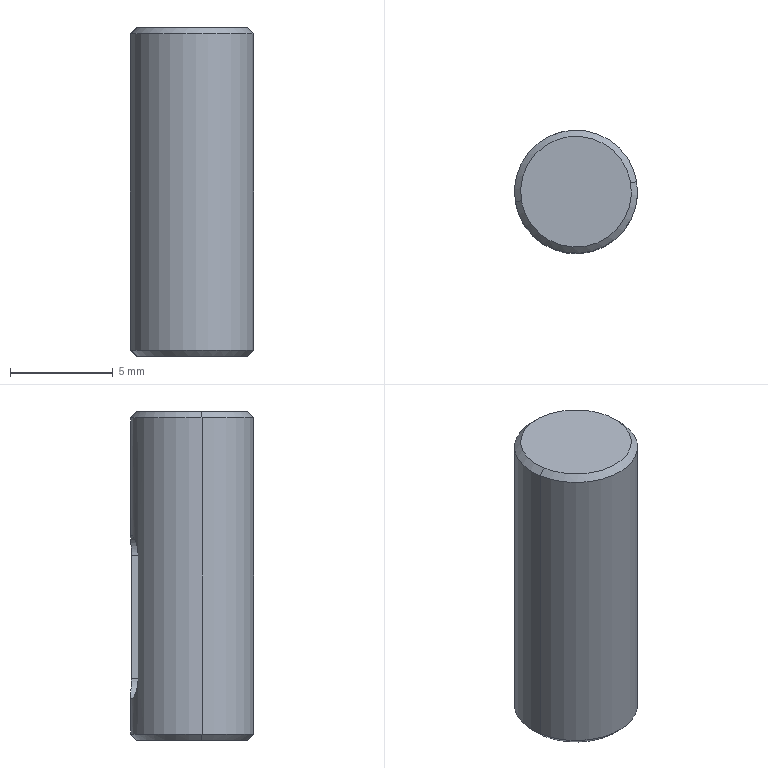Component | SolidWorks | GMotorAxis-1 | 1 solid | 17 faces | box 6 x 6 x 16 mm | volume 338 mm3 | cylinder 7 | plane 6 | cone 4 | commonest cylinder face diameters 2 x3 5.02 x2 6 x2
STEP:
#1=COLOUR_RGB('',0.7922,0.8196,0.9333);
#2=FILL_AREA_STYLE_COLOUR('',#1);
#3=FILL_AREA_STYLE('',(#2));
#4=SURFACE_STYLE_FILL_AREA(#3);
#5=SURFACE_SIDE_STYLE('',(#4));
#6=SURFACE_STYLE_USAGE(.BOTH.,#5);
#7=PRESENTATION_STYLE_ASSIGNMENT((#6));
#8=CARTESIAN_POINT('',(-0.5296,-0.05087,0.6339));
#9=VERTEX_POINT('',#8);
#10=CARTESIAN_POINT('',(-0.7246,-0.083,0.6339));
#11=VERTEX_POINT('',#10);
#12=CARTESIAN_POINT('',(-0.6271,-0.06694,0.6339));
#13=DIRECTION('',(0.,0.,-1.));
#14=DIRECTION('',(-0.9867,-0.1625,0.));
#15=AXIS2_PLACEMENT_3D('',#12,#13,#14);
#16=CIRCLE('',#15,0.09882);
#17=EDGE_CURVE('',#9,#11,#16,.T.);
#18=ORIENTED_EDGE('',*,*,#17,.F.);
#19=CARTESIAN_POINT('',(-0.5296,-0.05087,0.4331));
#20=VERTEX_POINT('',#19);
#21=CARTESIAN_POINT('',(-0.5296,-0.05087,0.6339));
#22=DIRECTION('',(0.,0.,-1.));
#23=VECTOR('',#22,39.37);
#24=LINE('',#21,#23);
#25=EDGE_CURVE('',#9,#20,#24,.T.);
#26=ORIENTED_EDGE('',*,*,#25,.T.);
#27=CARTESIAN_POINT('',(-0.7246,-0.083,0.4331));
#28=VERTEX_POINT('',#27);
#29=CARTESIAN_POINT('',(-0.6271,-0.06694,0.4331));
#30=DIRECTION('',(0.,0.,1.));
#31=DIRECTION('',(0.9867,0.1625,0.));
#32=AXIS2_PLACEMENT_3D('',#29,#30,#31);
#33=CIRCLE('',#32,0.09882);
#34=EDGE_CURVE('',#28,#20,#33,.T.);
#35=ORIENTED_EDGE('',*,*,#34,.F.);
#36=CARTESIAN_POINT('',(-0.7246,-0.083,0.6339));
#37=DIRECTION('',(0.,0.,-1.));
#38=VECTOR('',#37,39.37);
#39=LINE('',#36,#38);
#40=EDGE_CURVE('',#11,#28,#39,.T.);
#41=ORIENTED_EDGE('',*,*,#40,.F.);
#42=EDGE_LOOP('',(#18,#26,#35,#41));
#43=FACE_OUTER_BOUND('',#42,.T.);
#44=CARTESIAN_POINT('',(-0.6271,-0.06694,0.6339));
#45=DIRECTION('',(0.,0.,-1.));
#46=DIRECTION('',(-0.9867,-0.1625,0.));
#47=AXIS2_PLACEMENT_3D('',#44,#45,#46);
#48=CYLINDRICAL_SURFACE('',#47,0.09882);
#49=ADVANCED_FACE('',(#43),#48,.F.);
#50=CARTESIAN_POINT('',(-0.732,-0.08421,0.4331));
#51=VERTEX_POINT('',#50);
#52=CARTESIAN_POINT('',(-0.5222,-0.04966,0.4331));
#53=VERTEX_POINT('',#52);
#54=CARTESIAN_POINT('',(-0.6271,-0.06694,0.4331));
#55=DIRECTION('',(0.,0.,-1.));
#56=DIRECTION('',(0.9867,0.1625,0.));
#57=AXIS2_PLACEMENT_3D('',#54,#55,#56);
#58=CIRCLE('',#57,0.1063);
#59=EDGE_CURVE('',#51,#53,#58,.T.);
#60=ORIENTED_EDGE('',*,*,#59,.F.);
#61=CARTESIAN_POINT('',(-0.7436,-0.08613,0.4449));
#62=VERTEX_POINT('',#61);
#63=CARTESIAN_POINT('',(-0.7436,-0.08613,0.4449));
#64=DIRECTION('',(-0.6977,-0.1149,0.7071));
#65=VECTOR('',#64,39.37);
#66=LINE('',#63,#65);
#67=EDGE_CURVE('',#51,#62,#66,.T.);
#68=ORIENTED_EDGE('',*,*,#67,.T.);
#69=CARTESIAN_POINT('',(-0.5105,-0.04774,0.4449));
#70=VERTEX_POINT('',#69);
#71=CARTESIAN_POINT('',(-0.6271,-0.06694,0.4449));
#72=DIRECTION('',(0.,0.,1.));
#73=DIRECTION('',(0.9867,0.1625,0.));
#74=AXIS2_PLACEMENT_3D('',#71,#72,#73);
#75=CIRCLE('',#74,0.1181);
#76=EDGE_CURVE('',#70,#62,#75,.T.);
#77=ORIENTED_EDGE('',*,*,#76,.F.);
#78=CARTESIAN_POINT('',(-0.5105,-0.04774,0.4449));
#79=DIRECTION('',(0.6977,0.1149,0.7071));
#80=VECTOR('',#79,39.37);
#81=LINE('',#78,#80);
#82=EDGE_CURVE('',#53,#70,#81,.T.);
#83=ORIENTED_EDGE('',*,*,#82,.F.);
#84=EDGE_LOOP('',(#60,#68,#77,#83));
#85=FACE_OUTER_BOUND('',#84,.T.);
#86=CARTESIAN_POINT('',(-0.6271,-0.06694,0.4449));
#87=DIRECTION('',(0.,0.,1.));
#88=DIRECTION('',(0.9867,0.1625,0.));
#89=AXIS2_PLACEMENT_3D('',#86,#87,#88);
#90=CONICAL_SURFACE('',#89,0.1181,0.7854);
#91=ADVANCED_FACE('',(#85),#90,.T.);
#92=CARTESIAN_POINT('',(-0.5222,-0.04966,1.063));
#93=VERTEX_POINT('',#92);
#94=CARTESIAN_POINT('',(-0.732,-0.08421,1.063));
#95=VERTEX_POINT('',#94);
#96=CARTESIAN_POINT('',(-0.6271,-0.06694,1.063));
#97=DIRECTION('',(0.,0.,1.));
#98=DIRECTION('',(0.9867,0.1625,0.));
#99=AXIS2_PLACEMENT_3D('',#96,#97,#98);
#100=CIRCLE('',#99,0.1063);
#101=EDGE_CURVE('',#93,#95,#100,.T.);
#102=ORIENTED_EDGE('',*,*,#101,.F.);
#103=CARTESIAN_POINT('',(-0.5105,-0.04774,1.051));
#104=VERTEX_POINT('',#103);
#105=CARTESIAN_POINT('',(-0.5222,-0.04966,1.063));
#106=DIRECTION('',(0.6977,0.1149,-0.7071));
#107=VECTOR('',#106,39.37);
#108=LINE('',#105,#107);
#109=EDGE_CURVE('',#93,#104,#108,.T.);
#110=ORIENTED_EDGE('',*,*,#109,.T.);
#111=CARTESIAN_POINT('',(-0.7436,-0.08613,1.051));
#112=VERTEX_POINT('',#111);
#113=CARTESIAN_POINT('',(-0.6271,-0.06694,1.051));
#114=DIRECTION('',(0.,0.,-1.));
#115=DIRECTION('',(0.9867,0.1625,0.));
#116=AXIS2_PLACEMENT_3D('',#113,#114,#115);
#117=CIRCLE('',#116,0.1181);
#118=EDGE_CURVE('',#112,#104,#117,.T.);
#119=ORIENTED_EDGE('',*,*,#118,.F.);
#120=CARTESIAN_POINT('',(-0.732,-0.08421,1.063));
#121=DIRECTION('',(-0.6977,-0.1149,-0.7071));
#122=VECTOR('',#121,39.37);
#123=LINE('',#120,#122);
#124=EDGE_CURVE('',#95,#112,#123,.T.);
#125=ORIENTED_EDGE('',*,*,#124,.F.);
#126=EDGE_LOOP('',(#102,#110,#119,#125));
#127=FACE_OUTER_BOUND('',#126,.T.);
#128=CARTESIAN_POINT('',(-0.6271,-0.06694,1.063));
#129=DIRECTION('',(0.,0.,-1.));
#130=DIRECTION('',(-0.9867,-0.1625,0.));
#131=AXIS2_PLACEMENT_3D('',#128,#129,#130);
#132=CONICAL_SURFACE('',#131,0.1063,0.7854);
#133=ADVANCED_FACE('',(#127),#132,.T.);
#134=CARTESIAN_POINT('',(-0.684,0.03654,0.7874));
#135=VERTEX_POINT('',#134);
#136=CARTESIAN_POINT('',(-0.6463,0.0496,0.8268));
#137=VERTEX_POINT('',#136);
#138=CARTESIAN_POINT('',(-0.684,0.03654,0.7874));
#139=CARTESIAN_POINT('',(-0.684,0.03654,0.7926));
#140=CARTESIAN_POINT('',(-0.683,0.0371,0.7978));
#141=CARTESIAN_POINT('',(-0.6794,0.039,0.8073));
#142=CARTESIAN_POINT('',(-0.6766,0.04035,0.8116));
#143=CARTESIAN_POINT('',(-0.6698,0.04324,0.8188));
#144=CARTESIAN_POINT('',(-0.6657,0.0448,0.8218));
#145=CARTESIAN_POINT('',(-0.6565,0.04756,0.8257));
#146=CARTESIAN_POINT('',(-0.6515,0.04875,0.8268));
#147=CARTESIAN_POINT('',(-0.6463,0.0496,0.8268));
#148=B_SPLINE_CURVE_WITH_KNOTS('',3,(#138,#139,#140,#141,#142,#143,#144,#145,#146,#147),.UNSPECIFIED.,.F.,.F.,(4,2,2,2,4),(0.,0.000396,0.0007919,0.001188,0.001584),.UNSPECIFIED.);
#149=EDGE_CURVE('',#135,#137,#148,.T.);
#150=ORIENTED_EDGE('',*,*,#149,.F.);
#151=CARTESIAN_POINT('',(-0.684,0.03654,0.5512));
#152=VERTEX_POINT('',#151);
#153=CARTESIAN_POINT('',(-0.684,0.03654,1.063));
#154=DIRECTION('',(0.,0.,-1.));
#155=VECTOR('',#154,39.37);
#156=LINE('',#153,#155);
#157=EDGE_CURVE('',#135,#152,#156,.T.);
#158=ORIENTED_EDGE('',*,*,#157,.T.);
#159=CARTESIAN_POINT('',(-0.6063,0.04934,0.5512));
#160=VERTEX_POINT('',#159);
#161=CARTESIAN_POINT('',(-0.6063,0.04934,0.5512));
#162=CARTESIAN_POINT('',(-0.6063,0.04934,0.5459));
#163=CARTESIAN_POINT('',(-0.6075,0.04955,0.5407));
#164=CARTESIAN_POINT('',(-0.6116,0.05017,0.5313));
#165=CARTESIAN_POINT('',(-0.6146,0.05057,0.5269));
#166=CARTESIAN_POINT('',(-0.622,0.05112,0.5197));
#167=CARTESIAN_POINT('',(-0.6264,0.05127,0.5168));
#168=CARTESIAN_POINT('',(-0.636,0.05094,0.5129));
#169=CARTESIAN_POINT('',(-0.6411,0.05045,0.5118));
#170=CARTESIAN_POINT('',(-0.6515,0.04875,0.5118));
#171=CARTESIAN_POINT('',(-0.6565,0.04755,0.5129));
#172=CARTESIAN_POINT('',(-0.6657,0.0448,0.5168));
#173=CARTESIAN_POINT('',(-0.6698,0.04324,0.5197));
#174=CARTESIAN_POINT('',(-0.6766,0.04034,0.527));
#175=CARTESIAN_POINT('',(-0.6794,0.03899,0.5313));
#176=CARTESIAN_POINT('',(-0.6831,0.03709,0.5408));
#177=CARTESIAN_POINT('',(-0.684,0.03654,0.5459));
#178=CARTESIAN_POINT('',(-0.684,0.03654,0.5512));
#179=B_SPLINE_CURVE_WITH_KNOTS('',3,(#161,#162,#163,#164,#165,#166,#167,#168,#169,#170,#171,#172,#173,#174,#175,#176,#177,#178),.UNSPECIFIED.,.F.,.F.,(4,2,2,2,2,2,2,2,4),(0.,0.000396,0.0007919,0.001188,0.001584,0.00198,0.002376,0.002772,0.003168),.UNSPECIFIED.);
#180=EDGE_CURVE('',#160,#152,#179,.T.);
#181=ORIENTED_EDGE('',*,*,#180,.F.);
#182=CARTESIAN_POINT('',(-0.6063,0.04934,0.7874));
#183=VERTEX_POINT('',#182);
#184=CARTESIAN_POINT('',(-0.6063,0.04934,1.063));
#185=DIRECTION('',(0.,0.,1.));
#186=VECTOR('',#185,39.37);
#187=LINE('',#184,#186);
#188=EDGE_CURVE('',#160,#183,#187,.T.);
#189=ORIENTED_EDGE('',*,*,#188,.T.);
#190=CARTESIAN_POINT('',(-0.6463,0.0496,0.8268));
#191=CARTESIAN_POINT('',(-0.6411,0.05045,0.8268));
#192=CARTESIAN_POINT('',(-0.6359,0.05094,0.8257));
#193=CARTESIAN_POINT('',(-0.6264,0.05127,0.8218));
#194=CARTESIAN_POINT('',(-0.622,0.05112,0.8188));
#195=CARTESIAN_POINT('',(-0.6146,0.05057,0.8116));
#196=CARTESIAN_POINT('',(-0.6115,0.05017,0.8073));
#197=CARTESIAN_POINT('',(-0.6074,0.04955,0.7978));
#198=CARTESIAN_POINT('',(-0.6063,0.04934,0.7926));
#199=CARTESIAN_POINT('',(-0.6063,0.04934,0.7874));
#200=B_SPLINE_CURVE_WITH_KNOTS('',3,(#190,#191,#192,#193,#194,#195,#196,#197,#198,#199),.UNSPECIFIED.,.F.,.F.,(4,2,2,2,4),(0.001584,0.00198,0.002376,0.002772,0.003168),.UNSPECIFIED.);
#201=EDGE_CURVE('',#137,#183,#200,.T.);
#202=ORIENTED_EDGE('',*,*,#201,.F.);
#203=EDGE_LOOP('',(#150,#158,#181,#189,#202));
#204=FACE_BOUND('',#203,.T.);
#205=ORIENTED_EDGE('',*,*,#118,.T.);
#206=CARTESIAN_POINT('',(-0.5105,-0.04774,1.063));
#207=DIRECTION('',(0.,0.,-1.));
#208=VECTOR('',#207,39.37);
#209=LINE('',#206,#208);
#210=EDGE_CURVE('',#104,#70,#209,.T.);
#211=ORIENTED_EDGE('',*,*,#210,.T.);
#212=ORIENTED_EDGE('',*,*,#76,.T.);
#213=CARTESIAN_POINT('',(-0.7436,-0.08613,1.063));
#214=DIRECTION('',(0.,0.,-1.));
#215=VECTOR('',#214,39.37);
#216=LINE('',#213,#215);
#217=EDGE_CURVE('',#112,#62,#216,.T.);
#218=ORIENTED_EDGE('',*,*,#217,.F.);
#219=EDGE_LOOP('',(#205,#211,#212,#218));
#220=FACE_OUTER_BOUND('',#219,.T.);
#221=CARTESIAN_POINT('',(-0.6271,-0.06694,1.063));
#222=DIRECTION('',(0.,0.,-1.));
#223=DIRECTION('',(-0.9867,-0.1625,0.));
#224=AXIS2_PLACEMENT_3D('',#221,#222,#223);
#225=CYLINDRICAL_SURFACE('',#224,0.1181);
#226=ADVANCED_FACE('',(#204,#220),#225,.T.);
#227=CARTESIAN_POINT('',(-0.6399,0.01076,0.8268));
#228=VERTEX_POINT('',#227);
#229=CARTESIAN_POINT('',(-0.601,0.01716,0.7874));
#230=VERTEX_POINT('',#229);
#231=CARTESIAN_POINT('',(-0.6399,0.01076,0.7874));
#232=DIRECTION('',(-0.1625,0.9867,0.));
#233=DIRECTION('',(0.,0.,-1.));
#234=AXIS2_PLACEMENT_3D('',#231,#232,#233);
#235=CIRCLE('',#234,0.03937);
#236=EDGE_CURVE('',#228,#230,#235,.T.);
#237=ORIENTED_EDGE('',*,*,#236,.F.);
#238=CARTESIAN_POINT('',(-0.6452,0.04294,0.8268));
#239=DIRECTION('',(-0.1625,0.9867,0.));
#240=VECTOR('',#239,39.37);
#241=LINE('',#238,#240);
#242=EDGE_CURVE('',#228,#137,#241,.T.);
#243=ORIENTED_EDGE('',*,*,#242,.T.);
#244=ORIENTED_EDGE('',*,*,#201,.T.);
#245=CARTESIAN_POINT('',(-0.6063,0.04934,0.7874));
#246=DIRECTION('',(-0.1625,0.9867,0.));
#247=VECTOR('',#246,39.37);
#248=LINE('',#245,#247);
#249=EDGE_CURVE('',#230,#183,#248,.T.);
#250=ORIENTED_EDGE('',*,*,#249,.F.);
#251=EDGE_LOOP('',(#237,#243,#244,#250));
#252=FACE_OUTER_BOUND('',#251,.T.);
#253=CARTESIAN_POINT('',(-0.6452,0.04294,0.7874));
#254=DIRECTION('',(-0.1625,0.9867,0.));
#255=DIRECTION('',(0.,0.,1.));
#256=AXIS2_PLACEMENT_3D('',#253,#254,#255);
#257=CYLINDRICAL_SURFACE('',#256,0.03937);
#258=ADVANCED_FACE('',(#252),#257,.F.);
#259=CARTESIAN_POINT('',(-0.6787,0.004358,0.6339));
#260=VERTEX_POINT('',#259);
#261=CARTESIAN_POINT('',(-0.601,0.01716,0.6339));
#262=VERTEX_POINT('',#261);
#263=CARTESIAN_POINT('',(-0.6399,0.01076,0.6339));
#264=DIRECTION('',(0.9867,0.1625,0.));
#265=VECTOR('',#264,39.37);
#266=LINE('',#263,#265);
#267=EDGE_CURVE('',#260,#262,#266,.T.);
#268=ORIENTED_EDGE('',*,*,#267,.F.);
#269=CARTESIAN_POINT('',(-0.6787,0.004358,0.7874));
#270=VERTEX_POINT('',#269);
#271=CARTESIAN_POINT('',(-0.6787,0.004358,0.5118));
#272=DIRECTION('',(0.,0.,1.));
#273=VECTOR('',#272,39.37);
#274=LINE('',#271,#273);
#275=EDGE_CURVE('',#260,#270,#274,.T.);
#276=ORIENTED_EDGE('',*,*,#275,.T.);
#277=CARTESIAN_POINT('',(-0.6399,0.01076,0.7874));
#278=DIRECTION('',(-0.1625,0.9867,0.));
#279=DIRECTION('',(0.,0.,-1.));
#280=AXIS2_PLACEMENT_3D('',#277,#278,#279);
#281=CIRCLE('',#280,0.03937);
#282=EDGE_CURVE('',#270,#228,#281,.T.);
#283=ORIENTED_EDGE('',*,*,#282,.T.);
#284=ORIENTED_EDGE('',*,*,#236,.T.);
#285=CARTESIAN_POINT('',(-0.601,0.01716,0.5118));
#286=DIRECTION('',(-0.,-0.,-1.));
#287=VECTOR('',#286,39.37);
#288=LINE('',#285,#287);
#289=EDGE_CURVE('',#230,#262,#288,.T.);
#290=ORIENTED_EDGE('',*,*,#289,.T.);
#291=EDGE_LOOP('',(#268,#276,#283,#284,#290));
#292=FACE_OUTER_BOUND('',#291,.T.);
#293=CARTESIAN_POINT('',(-0.6399,0.01076,0.4331));
#294=DIRECTION('',(0.1625,-0.9867,0.));
#295=DIRECTION('',(0.,0.,-1.));
#296=AXIS2_PLACEMENT_3D('',#293,#294,#295);
#297=PLANE('',#296);
#298=ADVANCED_FACE('',(#292),#297,.F.);
#299=ORIENTED_EDGE('',*,*,#242,.F.);
#300=ORIENTED_EDGE('',*,*,#282,.F.);
#301=CARTESIAN_POINT('',(-0.684,0.03654,0.7874));
#302=DIRECTION('',(0.1625,-0.9867,0.));
#303=VECTOR('',#302,39.37);
#304=LINE('',#301,#303);
#305=EDGE_CURVE('',#135,#270,#304,.T.);
#306=ORIENTED_EDGE('',*,*,#305,.F.);
#307=ORIENTED_EDGE('',*,*,#149,.T.);
#308=EDGE_LOOP('',(#299,#300,#306,#307));
#309=FACE_OUTER_BOUND('',#308,.T.);
#310=CARTESIAN_POINT('',(-0.6452,0.04294,0.7874));
#311=DIRECTION('',(-0.1625,0.9867,0.));
#312=DIRECTION('',(0.,0.,1.));
#313=AXIS2_PLACEMENT_3D('',#310,#311,#312);
#314=CYLINDRICAL_SURFACE('',#313,0.03937);
#315=ADVANCED_FACE('',(#309),#314,.F.);
#316=CARTESIAN_POINT('',(-0.6807,0.0161,0.5512));
#317=VERTEX_POINT('',#316);
#318=CARTESIAN_POINT('',(-0.6787,0.004358,0.5512));
#319=DIRECTION('',(-0.1625,0.9867,0.));
#320=VECTOR('',#319,39.37);
#321=LINE('',#318,#320);
#322=EDGE_CURVE('',#317,#152,#321,.T.);
#323=ORIENTED_EDGE('',*,*,#322,.F.);
#324=CARTESIAN_POINT('',(-0.603,0.02889,0.5512));
#325=VERTEX_POINT('',#324);
#326=CARTESIAN_POINT('',(-0.6807,0.0161,0.5512));
#327=CARTESIAN_POINT('',(-0.6807,0.0161,0.5459));
#328=CARTESIAN_POINT('',(-0.6797,0.01674,0.5408));
#329=CARTESIAN_POINT('',(-0.676,0.01893,0.5313));
#330=CARTESIAN_POINT('',(-0.6733,0.02047,0.5269));
#331=CARTESIAN_POINT('',(-0.6666,0.02371,0.5198));
#332=CARTESIAN_POINT('',(-0.6625,0.02545,0.5168));
#333=CARTESIAN_POINT('',(-0.6534,0.02844,0.5129));
#334=CARTESIAN_POINT('',(-0.6483,0.02971,0.5118));
#335=CARTESIAN_POINT('',(-0.6381,0.03141,0.5118));
#336=CARTESIAN_POINT('',(-0.6329,0.03183,0.5128));
#337=CARTESIAN_POINT('',(-0.6232,0.03192,0.5168));
#338=CARTESIAN_POINT('',(-0.6188,0.0316,0.5197));
#339=CARTESIAN_POINT('',(-0.6113,0.03069,0.5269));
#340=CARTESIAN_POINT('',(-0.6083,0.0301,0.5313));
#341=CARTESIAN_POINT('',(-0.6041,0.0292,0.5407));
#342=CARTESIAN_POINT('',(-0.603,0.02889,0.5459));
#343=CARTESIAN_POINT('',(-0.603,0.02889,0.5512));
#344=B_SPLINE_CURVE_WITH_KNOTS('',3,(#326,#327,#328,#329,#330,#331,#332,#333,#334,#335,#336,#337,#338,#339,#340,#341,#342,#343),.UNSPECIFIED.,.F.,.F.,(4,2,2,2,2,2,2,2,4),(0.,0.0003948,0.0007895,0.001184,0.001579,0.001974,0.002369,0.002763,0.003158),.UNSPECIFIED.);
#345=EDGE_CURVE('',#317,#325,#344,.T.);
#346=ORIENTED_EDGE('',*,*,#345,.T.);
#347=CARTESIAN_POINT('',(-0.601,0.01716,0.5512));
#348=DIRECTION('',(0.1625,-0.9867,0.));
#349=VECTOR('',#348,39.37);
#350=LINE('',#347,#349);
#351=EDGE_CURVE('',#160,#325,#350,.T.);
#352=ORIENTED_EDGE('',*,*,#351,.F.);
#353=ORIENTED_EDGE('',*,*,#180,.T.);
#354=EDGE_LOOP('',(#323,#346,#352,#353));
#355=FACE_OUTER_BOUND('',#354,.T.);
#356=CARTESIAN_POINT('',(-0.6399,0.01076,0.5512));
#357=DIRECTION('',(-0.1625,0.9867,0.));
#358=DIRECTION('',(0.,0.,1.));
#359=AXIS2_PLACEMENT_3D('',#356,#357,#358);
#360=CYLINDRICAL_SURFACE('',#359,0.03937);
#361=ADVANCED_FACE('',(#355),#360,.F.);
#362=ORIENTED_EDGE('',*,*,#210,.F.);
#363=CARTESIAN_POINT('',(-0.6271,-0.06694,1.051));
#364=DIRECTION('',(0.,0.,-1.));
#365=DIRECTION('',(0.9867,0.1625,0.));
#366=AXIS2_PLACEMENT_3D('',#363,#364,#365);
#367=CIRCLE('',#366,0.1181);
#368=EDGE_CURVE('',#104,#112,#367,.T.);
#369=ORIENTED_EDGE('',*,*,#368,.T.);
#370=ORIENTED_EDGE('',*,*,#217,.T.);
#371=CARTESIAN_POINT('',(-0.6271,-0.06694,0.4449));
#372=DIRECTION('',(0.,0.,1.));
#373=DIRECTION('',(0.9867,0.1625,0.));
#374=AXIS2_PLACEMENT_3D('',#371,#372,#373);
#375=CIRCLE('',#374,0.1181);
#376=EDGE_CURVE('',#62,#70,#375,.T.);
#377=ORIENTED_EDGE('',*,*,#376,.T.);
#378=EDGE_LOOP('',(#362,#369,#370,#377));
#379=FACE_OUTER_BOUND('',#378,.T.);
#380=CARTESIAN_POINT('',(-0.6271,-0.06694,1.063));
#381=DIRECTION('',(0.,0.,-1.));
#382=DIRECTION('',(-0.9867,-0.1625,0.));
#383=AXIS2_PLACEMENT_3D('',#380,#381,#382);
#384=CYLINDRICAL_SURFACE('',#383,0.1181);
#385=ADVANCED_FACE('',(#379),#384,.T.);
#386=CARTESIAN_POINT('',(-0.6271,-0.06694,1.063));
#387=DIRECTION('',(0.,0.,1.));
#388=DIRECTION('',(0.9867,0.1625,0.));
#389=AXIS2_PLACEMENT_3D('',#386,#387,#388);
#390=CIRCLE('',#389,0.1063);
#391=EDGE_CURVE('',#95,#93,#390,.T.);
#392=ORIENTED_EDGE('',*,*,#391,.T.);
#393=ORIENTED_EDGE('',*,*,#101,.T.);
#394=EDGE_LOOP('',(#392,#393));
#395=FACE_OUTER_BOUND('',#394,.T.);
#396=CARTESIAN_POINT('',(-0.6271,-0.06694,1.063));
#397=DIRECTION('',(0.,0.,1.));
#398=DIRECTION('',(0.9867,0.1625,0.));
#399=AXIS2_PLACEMENT_3D('',#396,#397,#398);
#400=PLANE('',#399);
#401=ADVANCED_FACE('',(#395),#400,.T.);
#402=ORIENTED_EDGE('',*,*,#34,.T.);
#403=CARTESIAN_POINT('',(-0.6271,-0.06694,0.4331));
#404=DIRECTION('',(0.,0.,1.));
#405=DIRECTION('',(0.9867,0.1625,0.));
#406=AXIS2_PLACEMENT_3D('',#403,#404,#405);
#407=CIRCLE('',#406,0.09882);
#408=EDGE_CURVE('',#20,#28,#407,.T.);
#409=ORIENTED_EDGE('',*,*,#408,.T.);
#410=EDGE_LOOP('',(#402,#409));
#411=FACE_BOUND('',#410,.T.);
#412=CARTESIAN_POINT('',(-0.6271,-0.06694,0.4331));
#413=DIRECTION('',(0.,0.,-1.));
#414=DIRECTION('',(0.9867,0.1625,0.));
#415=AXIS2_PLACEMENT_3D('',#412,#413,#414);
#416=CIRCLE('',#415,0.1063);
#417=EDGE_CURVE('',#53,#51,#416,.T.);
#418=ORIENTED_EDGE('',*,*,#417,.T.);
#419=ORIENTED_EDGE('',*,*,#59,.T.);
#420=EDGE_LOOP('',(#418,#419));
#421=FACE_OUTER_BOUND('',#420,.T.);
#422=CARTESIAN_POINT('',(-0.6271,-0.06694,0.4331));
#423=DIRECTION('',(0.,0.,1.));
#424=DIRECTION('',(0.9867,0.1625,0.));
#425=AXIS2_PLACEMENT_3D('',#422,#423,#424);
#426=PLANE('',#425);
#427=ADVANCED_FACE('',(#411,#421),#426,.F.);
#428=CARTESIAN_POINT('',(-0.6807,0.0161,0.6339));
#429=VERTEX_POINT('',#428);
#430=CARTESIAN_POINT('',(-0.6787,0.004358,0.6339));
#431=DIRECTION('',(0.1625,-0.9867,0.));
#432=VECTOR('',#431,39.37);
#433=LINE('',#430,#432);
#434=EDGE_CURVE('',#429,#260,#433,.T.);
#435=ORIENTED_EDGE('',*,*,#434,.F.);
#436=CARTESIAN_POINT('',(-0.6807,0.0161,0.6339));
#437=DIRECTION('',(0.,0.,-1.));
#438=VECTOR('',#437,39.37);
#439=LINE('',#436,#438);
#440=EDGE_CURVE('',#429,#317,#439,.T.);
#441=ORIENTED_EDGE('',*,*,#440,.T.);
#442=ORIENTED_EDGE('',*,*,#322,.T.);
#443=ORIENTED_EDGE('',*,*,#157,.F.);
#444=ORIENTED_EDGE('',*,*,#305,.T.);
#445=ORIENTED_EDGE('',*,*,#275,.F.);
#446=EDGE_LOOP('',(#435,#441,#442,#443,#444,#445));
#447=FACE_OUTER_BOUND('',#446,.T.);
#448=CARTESIAN_POINT('',(-0.6787,0.004358,0.5118));
#449=DIRECTION('',(-0.9867,-0.1625,0.));
#450=DIRECTION('',(0.,0.,1.));
#451=AXIS2_PLACEMENT_3D('',#448,#449,#450);
#452=PLANE('',#451);
#453=ADVANCED_FACE('',(#447),#452,.F.);
#454=ORIENTED_EDGE('',*,*,#351,.T.);
#455=CARTESIAN_POINT('',(-0.603,0.02889,0.6339));
#456=VERTEX_POINT('',#455);
#457=CARTESIAN_POINT('',(-0.603,0.02889,0.6339));
#458=DIRECTION('',(0.,0.,1.));
#459=VECTOR('',#458,39.37);
#460=LINE('',#457,#459);
#461=EDGE_CURVE('',#325,#456,#460,.T.);
#462=ORIENTED_EDGE('',*,*,#461,.T.);
#463=CARTESIAN_POINT('',(-0.601,0.01716,0.6339));
#464=DIRECTION('',(-0.1625,0.9867,0.));
#465=VECTOR('',#464,39.37);
#466=LINE('',#463,#465);
#467=EDGE_CURVE('',#262,#456,#466,.T.);
#468=ORIENTED_EDGE('',*,*,#467,.F.);
#469=ORIENTED_EDGE('',*,*,#289,.F.);
#470=ORIENTED_EDGE('',*,*,#249,.T.);
#471=ORIENTED_EDGE('',*,*,#188,.F.);
#472=EDGE_LOOP('',(#454,#462,#468,#469,#470,#471));
#473=FACE_OUTER_BOUND('',#472,.T.);
#474=CARTESIAN_POINT('',(-0.601,0.01716,0.5118));
#475=DIRECTION('',(0.9867,0.1625,-0.));
#476=DIRECTION('',(-0.,-0.,-1.));
#477=AXIS2_PLACEMENT_3D('',#474,#475,#476);
#478=PLANE('',#477);
#479=ADVANCED_FACE('',(#473),#478,.F.);
#480=ORIENTED_EDGE('',*,*,#109,.F.);
#481=ORIENTED_EDGE('',*,*,#391,.F.);
#482=ORIENTED_EDGE('',*,*,#124,.T.);
#483=ORIENTED_EDGE('',*,*,#368,.F.);
#484=EDGE_LOOP('',(#480,#481,#482,#483));
#485=FACE_OUTER_BOUND('',#484,.T.);
#486=CARTESIAN_POINT('',(-0.6271,-0.06694,1.063));
#487=DIRECTION('',(0.,0.,-1.));
#488=DIRECTION('',(-0.9867,-0.1625,0.));
#489=AXIS2_PLACEMENT_3D('',#486,#487,#488);
#490=CONICAL_SURFACE('',#489,0.1063,0.7854);
#491=ADVANCED_FACE('',(#485),#490,.T.);
#492=ORIENTED_EDGE('',*,*,#67,.F.);
#493=ORIENTED_EDGE('',*,*,#417,.F.);
#494=ORIENTED_EDGE('',*,*,#82,.T.);
#495=ORIENTED_EDGE('',*,*,#376,.F.);
#496=EDGE_LOOP('',(#492,#493,#494,#495));
#497=FACE_OUTER_BOUND('',#496,.T.);
#498=CARTESIAN_POINT('',(-0.6271,-0.06694,0.4449));
#499=DIRECTION('',(0.,0.,1.));
#500=DIRECTION('',(0.9867,0.1625,0.));
#501=AXIS2_PLACEMENT_3D('',#498,#499,#500);
#502=CONICAL_SURFACE('',#501,0.1181,0.7854);
#503=ADVANCED_FACE('',(#497),#502,.T.);
#504=ORIENTED_EDGE('',*,*,#25,.F.);
#505=CARTESIAN_POINT('',(-0.6271,-0.06694,0.6339));
#506=DIRECTION('',(0.,0.,-1.));
#507=DIRECTION('',(-0.9867,-0.1625,0.));
#508=AXIS2_PLACEMENT_3D('',#505,#506,#507);
#509=CIRCLE('',#508,0.09882);
#510=EDGE_CURVE('',#456,#9,#509,.T.);
#511=ORIENTED_EDGE('',*,*,#510,.F.);
#512=ORIENTED_EDGE('',*,*,#461,.F.);
#513=ORIENTED_EDGE('',*,*,#345,.F.);
#514=ORIENTED_EDGE('',*,*,#440,.F.);
#515=CARTESIAN_POINT('',(-0.6271,-0.06694,0.6339));
#516=DIRECTION('',(0.,0.,-1.));
#517=DIRECTION('',(-0.9867,-0.1625,0.));
#518=AXIS2_PLACEMENT_3D('',#515,#516,#517);
#519=CIRCLE('',#518,0.09882);
#520=EDGE_CURVE('',#11,#429,#519,.T.);
#521=ORIENTED_EDGE('',*,*,#520,.F.);
#522=ORIENTED_EDGE('',*,*,#40,.T.);
#523=ORIENTED_EDGE('',*,*,#408,.F.);
#524=EDGE_LOOP('',(#504,#511,#512,#513,#514,#521,#522,#523));
#525=FACE_OUTER_BOUND('',#524,.T.);
#526=CARTESIAN_POINT('',(-0.6271,-0.06694,0.6339));
#527=DIRECTION('',(0.,0.,-1.));
#528=DIRECTION('',(-0.9867,-0.1625,0.));
#529=AXIS2_PLACEMENT_3D('',#526,#527,#528);
#530=CYLINDRICAL_SURFACE('',#529,0.09882);
#531=ADVANCED_FACE('',(#525),#530,.F.);
#532=ORIENTED_EDGE('',*,*,#434,.T.);
#533=ORIENTED_EDGE('',*,*,#267,.T.);
#534=ORIENTED_EDGE('',*,*,#467,.T.);
#535=ORIENTED_EDGE('',*,*,#510,.T.);
#536=ORIENTED_EDGE('',*,*,#17,.T.);
#537=ORIENTED_EDGE('',*,*,#520,.T.);
#538=EDGE_LOOP('',(#532,#533,#534,#535,#536,#537));
#539=FACE_OUTER_BOUND('',#538,.T.);
#540=CARTESIAN_POINT('',(-0.6271,-0.06694,0.6339));
#541=DIRECTION('',(0.,0.,-1.));
#542=DIRECTION('',(-0.9867,-0.1625,0.));
#543=AXIS2_PLACEMENT_3D('',#540,#541,#542);
#544=PLANE('',#543);
#545=ADVANCED_FACE('',(#539),#544,.T.);
#546=CLOSED_SHELL('',(#49,#91,#133,#226,#258,#298,#315,#361,#385,#401,#427,#453,#479,#491,#503,#531,#545));
#547=MANIFOLD_SOLID_BREP('',#546);
#548=STYLED_ITEM('',(#7),#547);
#549=(LENGTH_UNIT()NAMED_UNIT(*)SI_UNIT($,.METRE.));
#550=LENGTH_MEASURE_WITH_UNIT(LENGTH_MEASURE(0.0254),#549);
#551=DIMENSIONAL_EXPONENTS(1.,0.,0.,0.,0.,0.,0.);
#552=(CONVERSION_BASED_UNIT('',#550)LENGTH_UNIT()NAMED_UNIT(#551));
#553=UNCERTAINTY_MEASURE_WITH_UNIT(LENGTH_MEASURE(0.00001),#552,'','');
#554=(NAMED_UNIT(*)PLANE_ANGLE_UNIT()SI_UNIT($,.RADIAN.));
#555=(NAMED_UNIT(*)SI_UNIT($,.STERADIAN.)SOLID_ANGLE_UNIT());
#556=(GEOMETRIC_REPRESENTATION_CONTEXT(3)GLOBAL_UNCERTAINTY_ASSIGNED_CONTEXT((#553))GLOBAL_UNIT_ASSIGNED_CONTEXT((#552,#554,#555))REPRESENTATION_CONTEXT('',''));
#557=MECHANICAL_DESIGN_GEOMETRIC_PRESENTATION_REPRESENTATION('',(#548),#556);
#558=CARTESIAN_POINT('',(0.,0.,0.));
#559=DIRECTION('',(0.,0.,1.));
#560=DIRECTION('',(1.,0.,0.));
#561=AXIS2_PLACEMENT_3D('',#558,#559,#560);
#562=(LENGTH_UNIT()NAMED_UNIT(*)SI_UNIT($,.METRE.));
#563=LENGTH_MEASURE_WITH_UNIT(LENGTH_MEASURE(0.0254),#562);
#564=DIMENSIONAL_EXPONENTS(1.,0.,0.,0.,0.,0.,0.);
#565=(CONVERSION_BASED_UNIT('',#563)LENGTH_UNIT()NAMED_UNIT(#564));
#566=UNCERTAINTY_MEASURE_WITH_UNIT(LENGTH_MEASURE(0.00001),#565,'','');
#567=(NAMED_UNIT(*)PLANE_ANGLE_UNIT()SI_UNIT($,.RADIAN.));
#568=(NAMED_UNIT(*)SI_UNIT($,.STERADIAN.)SOLID_ANGLE_UNIT());
#569=(GEOMETRIC_REPRESENTATION_CONTEXT(3)GLOBAL_UNCERTAINTY_ASSIGNED_CONTEXT((#566))GLOBAL_UNIT_ASSIGNED_CONTEXT((#565,#567,#568))REPRESENTATION_CONTEXT('',''));
#570=ADVANCED_BREP_SHAPE_REPRESENTATION('',(#547,#561),#569);
#571=PRESENTATION_LAYER_ASSIGNMENT('','',(#548));